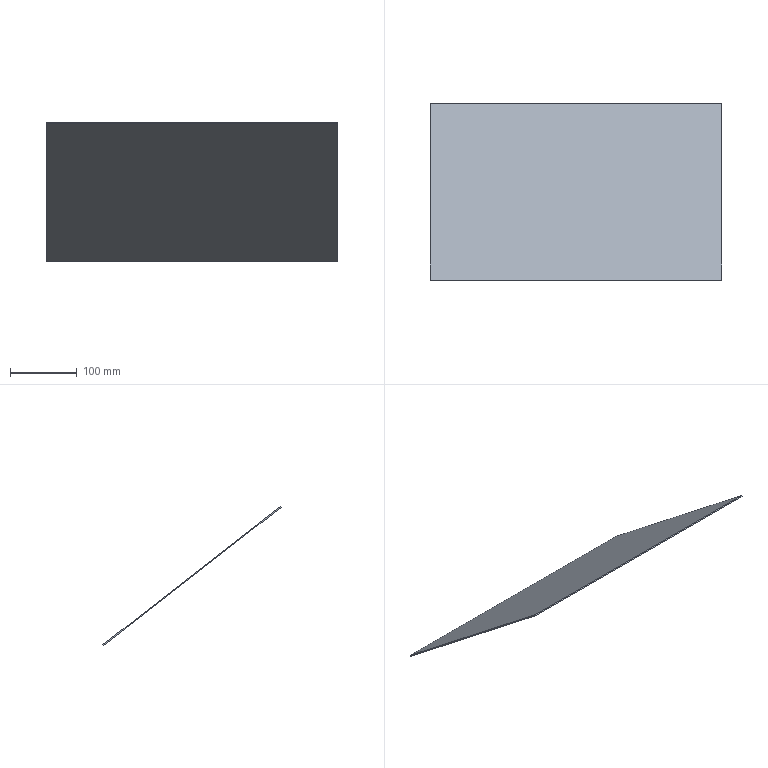Component | SolidWorks | DoorGlass-1 | 1 solid | 6 faces | box 438 x 267.58 x 209.67 mm | volume 296088 mm3 | plane 6 | material Plain Carbon Steel
build123d program:
from build123d import *

# Parameters (mm, degrees)
SKETCH1_W           = 438
SKETCH1_H           = 338
BOSS_EXTRUDE1_DEPTH = 2


with BuildPart() as part:
    # Sketch1 → Boss-Extrude1 (new body)
    with BuildSketch(Plane.XY):
        with Locations((87.682, -133.989)):
            Rectangle(SKETCH1_W, SKETCH1_H)
    extrude(amount=BOSS_EXTRUDE1_DEPTH)


solid = part.part

# Placed as in the assembly
solid = solid.moved(Location((-481.867, 78.402, 430.749), (-38, 0, 180)))
STEP:
#1=CARTESIAN_POINT('',(-31.045,12.487,9.615));
#2=VERTEX_POINT('',#1);
#3=CARTESIAN_POINT('',(-31.045,2.001,17.807));
#4=VERTEX_POINT('',#3);
#5=CARTESIAN_POINT('',(-31.045,12.487,9.615));
#6=DIRECTION('',(0.,-0.788,0.6157));
#7=VECTOR('',#6,39.37);
#8=LINE('',#5,#7);
#9=EDGE_CURVE('',#2,#4,#8,.T.);
#10=ORIENTED_EDGE('',*,*,#9,.T.);
#11=CARTESIAN_POINT('',(-31.045,2.049,17.869));
#12=VERTEX_POINT('',#11);
#13=CARTESIAN_POINT('',(-31.045,2.049,17.869));
#14=DIRECTION('',(-0.,-0.6157,-0.788));
#15=VECTOR('',#14,39.37);
#16=LINE('',#13,#15);
#17=EDGE_CURVE('',#12,#4,#16,.T.);
#18=ORIENTED_EDGE('',*,*,#17,.F.);
#19=CARTESIAN_POINT('',(-31.045,12.535,9.677));
#20=VERTEX_POINT('',#19);
#21=CARTESIAN_POINT('',(-31.045,12.535,9.677));
#22=DIRECTION('',(0.,-0.788,0.6157));
#23=VECTOR('',#22,39.37);
#24=LINE('',#21,#23);
#25=EDGE_CURVE('',#20,#12,#24,.T.);
#26=ORIENTED_EDGE('',*,*,#25,.F.);
#27=CARTESIAN_POINT('',(-31.045,12.535,9.677));
#28=DIRECTION('',(-0.,-0.6157,-0.788));
#29=VECTOR('',#28,39.37);
#30=LINE('',#27,#29);
#31=EDGE_CURVE('',#20,#2,#30,.T.);
#32=ORIENTED_EDGE('',*,*,#31,.T.);
#33=EDGE_LOOP('',(#10,#18,#26,#32));
#34=FACE_OUTER_BOUND('',#33,.T.);
#35=CARTESIAN_POINT('',(-31.045,12.535,9.677));
#36=DIRECTION('',(1.,0.,-0.));
#37=DIRECTION('',(-0.,0.788,-0.6157));
#38=AXIS2_PLACEMENT_3D('',#35,#36,#37);
#39=PLANE('',#38);
#40=ADVANCED_FACE('',(#34),#39,.F.);
#41=CARTESIAN_POINT('',(-13.801,2.001,17.807));
#42=VERTEX_POINT('',#41);
#43=CARTESIAN_POINT('',(-31.045,2.001,17.807));
#44=DIRECTION('',(1.,0.,-0.));
#45=VECTOR('',#44,39.37);
#46=LINE('',#43,#45);
#47=EDGE_CURVE('',#4,#42,#46,.T.);
#48=ORIENTED_EDGE('',*,*,#47,.T.);
#49=CARTESIAN_POINT('',(-13.801,2.049,17.869));
#50=VERTEX_POINT('',#49);
#51=CARTESIAN_POINT('',(-13.801,2.049,17.869));
#52=DIRECTION('',(-0.,-0.6157,-0.788));
#53=VECTOR('',#52,39.37);
#54=LINE('',#51,#53);
#55=EDGE_CURVE('',#50,#42,#54,.T.);
#56=ORIENTED_EDGE('',*,*,#55,.F.);
#57=CARTESIAN_POINT('',(-31.045,2.049,17.869));
#58=DIRECTION('',(1.,0.,-0.));
#59=VECTOR('',#58,39.37);
#60=LINE('',#57,#59);
#61=EDGE_CURVE('',#12,#50,#60,.T.);
#62=ORIENTED_EDGE('',*,*,#61,.F.);
#63=ORIENTED_EDGE('',*,*,#17,.T.);
#64=EDGE_LOOP('',(#48,#56,#62,#63));
#65=FACE_OUTER_BOUND('',#64,.T.);
#66=CARTESIAN_POINT('',(-31.045,2.049,17.869));
#67=DIRECTION('',(-0.,0.788,-0.6157));
#68=DIRECTION('',(0.,0.6157,0.788));
#69=AXIS2_PLACEMENT_3D('',#66,#67,#68);
#70=PLANE('',#69);
#71=ADVANCED_FACE('',(#65),#70,.F.);
#72=CARTESIAN_POINT('',(-13.801,12.487,9.615));
#73=VERTEX_POINT('',#72);
#74=CARTESIAN_POINT('',(-13.801,12.487,9.615));
#75=DIRECTION('',(-0.,0.788,-0.6157));
#76=VECTOR('',#75,39.37);
#77=LINE('',#74,#76);
#78=EDGE_CURVE('',#42,#73,#77,.T.);
#79=ORIENTED_EDGE('',*,*,#78,.T.);
#80=CARTESIAN_POINT('',(-13.801,12.535,9.677));
#81=VERTEX_POINT('',#80);
#82=CARTESIAN_POINT('',(-13.801,12.535,9.677));
#83=DIRECTION('',(-0.,-0.6157,-0.788));
#84=VECTOR('',#83,39.37);
#85=LINE('',#82,#84);
#86=EDGE_CURVE('',#81,#73,#85,.T.);
#87=ORIENTED_EDGE('',*,*,#86,.F.);
#88=CARTESIAN_POINT('',(-13.801,12.535,9.677));
#89=DIRECTION('',(-0.,0.788,-0.6157));
#90=VECTOR('',#89,39.37);
#91=LINE('',#88,#90);
#92=EDGE_CURVE('',#50,#81,#91,.T.);
#93=ORIENTED_EDGE('',*,*,#92,.F.);
#94=ORIENTED_EDGE('',*,*,#55,.T.);
#95=EDGE_LOOP('',(#79,#87,#93,#94));
#96=FACE_OUTER_BOUND('',#95,.T.);
#97=CARTESIAN_POINT('',(-13.801,12.535,9.677));
#98=DIRECTION('',(-1.,-0.,0.));
#99=DIRECTION('',(0.,-0.788,0.6157));
#100=AXIS2_PLACEMENT_3D('',#97,#98,#99);
#101=PLANE('',#100);
#102=ADVANCED_FACE('',(#96),#101,.F.);
#103=CARTESIAN_POINT('',(-31.045,12.487,9.615));
#104=DIRECTION('',(-1.,-0.,0.));
#105=VECTOR('',#104,39.37);
#106=LINE('',#103,#105);
#107=EDGE_CURVE('',#73,#2,#106,.T.);
#108=ORIENTED_EDGE('',*,*,#107,.T.);
#109=ORIENTED_EDGE('',*,*,#31,.F.);
#110=CARTESIAN_POINT('',(-31.045,12.535,9.677));
#111=DIRECTION('',(-1.,-0.,0.));
#112=VECTOR('',#111,39.37);
#113=LINE('',#110,#112);
#114=EDGE_CURVE('',#81,#20,#113,.T.);
#115=ORIENTED_EDGE('',*,*,#114,.F.);
#116=ORIENTED_EDGE('',*,*,#86,.T.);
#117=EDGE_LOOP('',(#108,#109,#115,#116));
#118=FACE_OUTER_BOUND('',#117,.T.);
#119=CARTESIAN_POINT('',(-31.045,12.535,9.677));
#120=DIRECTION('',(0.,-0.788,0.6157));
#121=DIRECTION('',(-0.,-0.6157,-0.788));
#122=AXIS2_PLACEMENT_3D('',#119,#120,#121);
#123=PLANE('',#122);
#124=ADVANCED_FACE('',(#118),#123,.F.);
#125=ORIENTED_EDGE('',*,*,#25,.T.);
#126=ORIENTED_EDGE('',*,*,#61,.T.);
#127=ORIENTED_EDGE('',*,*,#92,.T.);
#128=ORIENTED_EDGE('',*,*,#114,.T.);
#129=EDGE_LOOP('',(#125,#126,#127,#128));
#130=FACE_OUTER_BOUND('',#129,.T.);
#131=CARTESIAN_POINT('',(-25.875,11.449,10.525));
#132=DIRECTION('',(0.,0.6157,0.788));
#133=DIRECTION('',(1.,0.,-0.));
#134=AXIS2_PLACEMENT_3D('',#131,#132,#133);
#135=PLANE('',#134);
#136=ADVANCED_FACE('',(#130),#135,.T.);
#137=ORIENTED_EDGE('',*,*,#9,.F.);
#138=ORIENTED_EDGE('',*,*,#107,.F.);
#139=ORIENTED_EDGE('',*,*,#78,.F.);
#140=ORIENTED_EDGE('',*,*,#47,.F.);
#141=EDGE_LOOP('',(#137,#138,#139,#140));
#142=FACE_OUTER_BOUND('',#141,.T.);
#143=CARTESIAN_POINT('',(-25.875,11.4,10.463));
#144=DIRECTION('',(0.,0.6157,0.788));
#145=DIRECTION('',(1.,0.,-0.));
#146=AXIS2_PLACEMENT_3D('',#143,#144,#145);
#147=PLANE('',#146);
#148=ADVANCED_FACE('',(#142),#147,.F.);
#149=CLOSED_SHELL('',(#40,#71,#102,#124,#136,#148));
#150=MANIFOLD_SOLID_BREP('',#149);
#151=CARTESIAN_POINT('',(0.,0.,0.));
#152=DIRECTION('',(0.,0.,1.));
#153=DIRECTION('',(1.,0.,0.));
#154=AXIS2_PLACEMENT_3D('',#151,#152,#153);
#155=(LENGTH_UNIT()NAMED_UNIT(*)SI_UNIT($,.METRE.));
#156=LENGTH_MEASURE_WITH_UNIT(LENGTH_MEASURE(0.0254),#155);
#157=DIMENSIONAL_EXPONENTS(1.,0.,0.,0.,0.,0.,0.);
#158=(CONVERSION_BASED_UNIT('',#156)LENGTH_UNIT()NAMED_UNIT(#157));
#159=UNCERTAINTY_MEASURE_WITH_UNIT(LENGTH_MEASURE(0.00001),#158,'','');
#160=(NAMED_UNIT(*)PLANE_ANGLE_UNIT()SI_UNIT($,.RADIAN.));
#161=(NAMED_UNIT(*)SI_UNIT($,.STERADIAN.)SOLID_ANGLE_UNIT());
#162=(GEOMETRIC_REPRESENTATION_CONTEXT(3)GLOBAL_UNCERTAINTY_ASSIGNED_CONTEXT((#159))GLOBAL_UNIT_ASSIGNED_CONTEXT((#158,#160,#161))REPRESENTATION_CONTEXT('',''));
#163=ADVANCED_BREP_SHAPE_REPRESENTATION('',(#150,#154),#162);
#164=COLOUR_RGB('',0.7922,0.8196,0.9333);
#165=FILL_AREA_STYLE_COLOUR('',#164);
#166=FILL_AREA_STYLE('',(#165));
#167=SURFACE_STYLE_FILL_AREA(#166);
#168=SURFACE_SIDE_STYLE('',(#167));
#169=SURFACE_STYLE_USAGE(.BOTH.,#168);
#170=PRESENTATION_STYLE_ASSIGNMENT((#169));
#171=STYLED_ITEM('',(#170),#150);
#172=(LENGTH_UNIT()NAMED_UNIT(*)SI_UNIT($,.METRE.));
#173=LENGTH_MEASURE_WITH_UNIT(LENGTH_MEASURE(0.0254),#172);
#174=DIMENSIONAL_EXPONENTS(1.,0.,0.,0.,0.,0.,0.);
#175=(CONVERSION_BASED_UNIT('',#173)LENGTH_UNIT()NAMED_UNIT(#174));
#176=UNCERTAINTY_MEASURE_WITH_UNIT(LENGTH_MEASURE(0.00001),#175,'','');
#177=(NAMED_UNIT(*)PLANE_ANGLE_UNIT()SI_UNIT($,.RADIAN.));
#178=(NAMED_UNIT(*)SI_UNIT($,.STERADIAN.)SOLID_ANGLE_UNIT());
#179=(GEOMETRIC_REPRESENTATION_CONTEXT(3)GLOBAL_UNCERTAINTY_ASSIGNED_CONTEXT((#176))GLOBAL_UNIT_ASSIGNED_CONTEXT((#175,#177,#178))REPRESENTATION_CONTEXT('',''));
#180=MECHANICAL_DESIGN_GEOMETRIC_PRESENTATION_REPRESENTATION('',(#171),#179);
#181=PRESENTATION_LAYER_ASSIGNMENT('','',(#171));